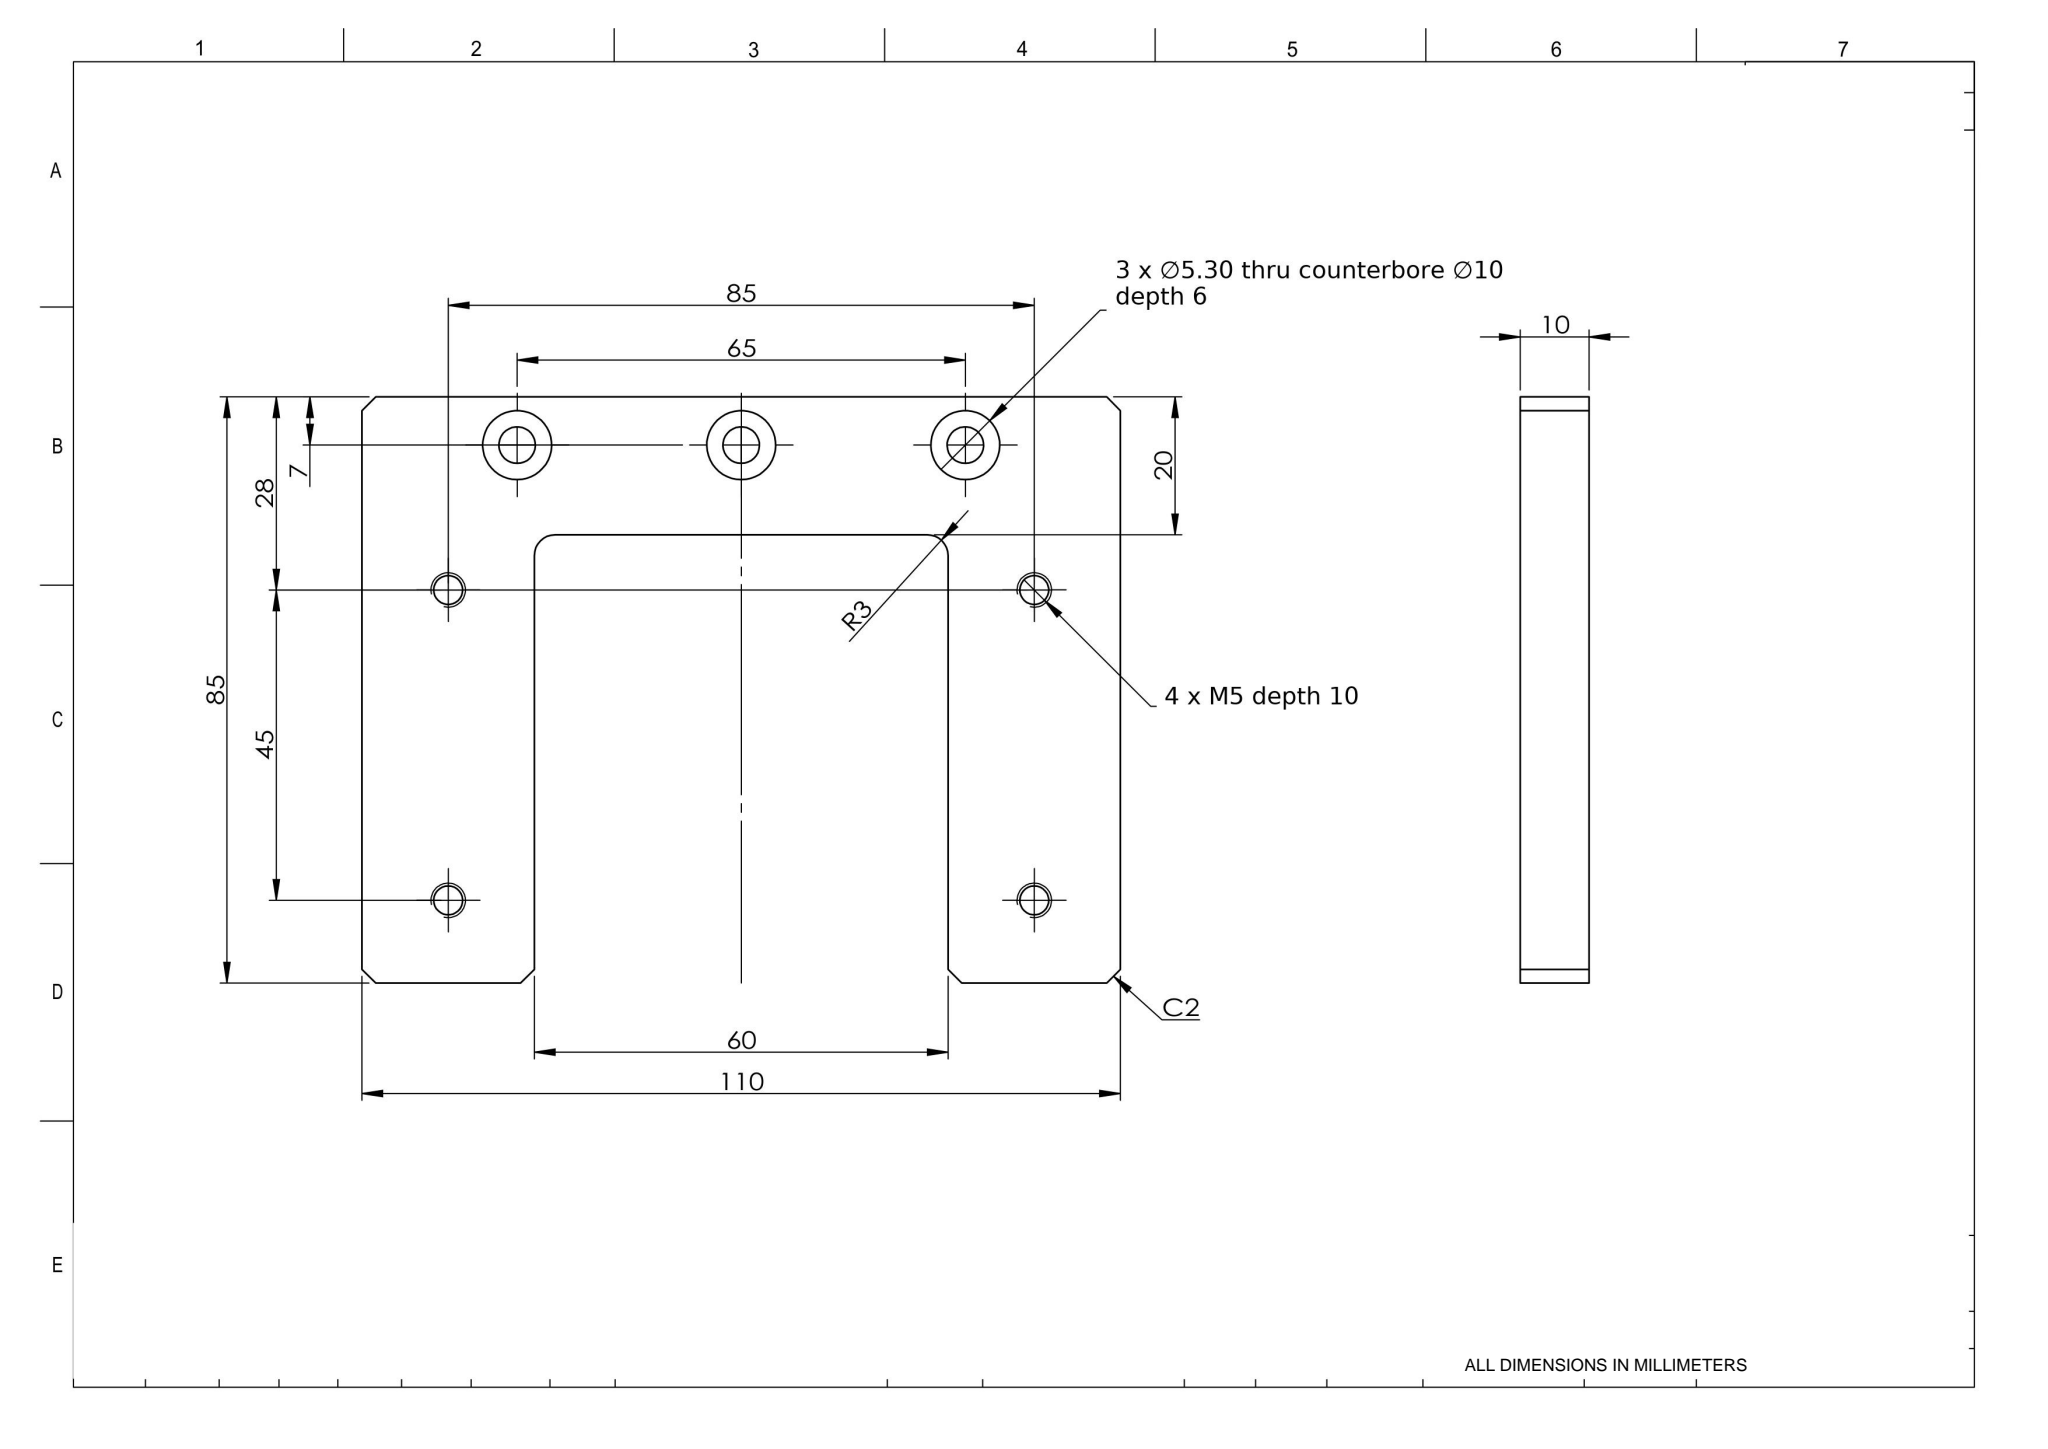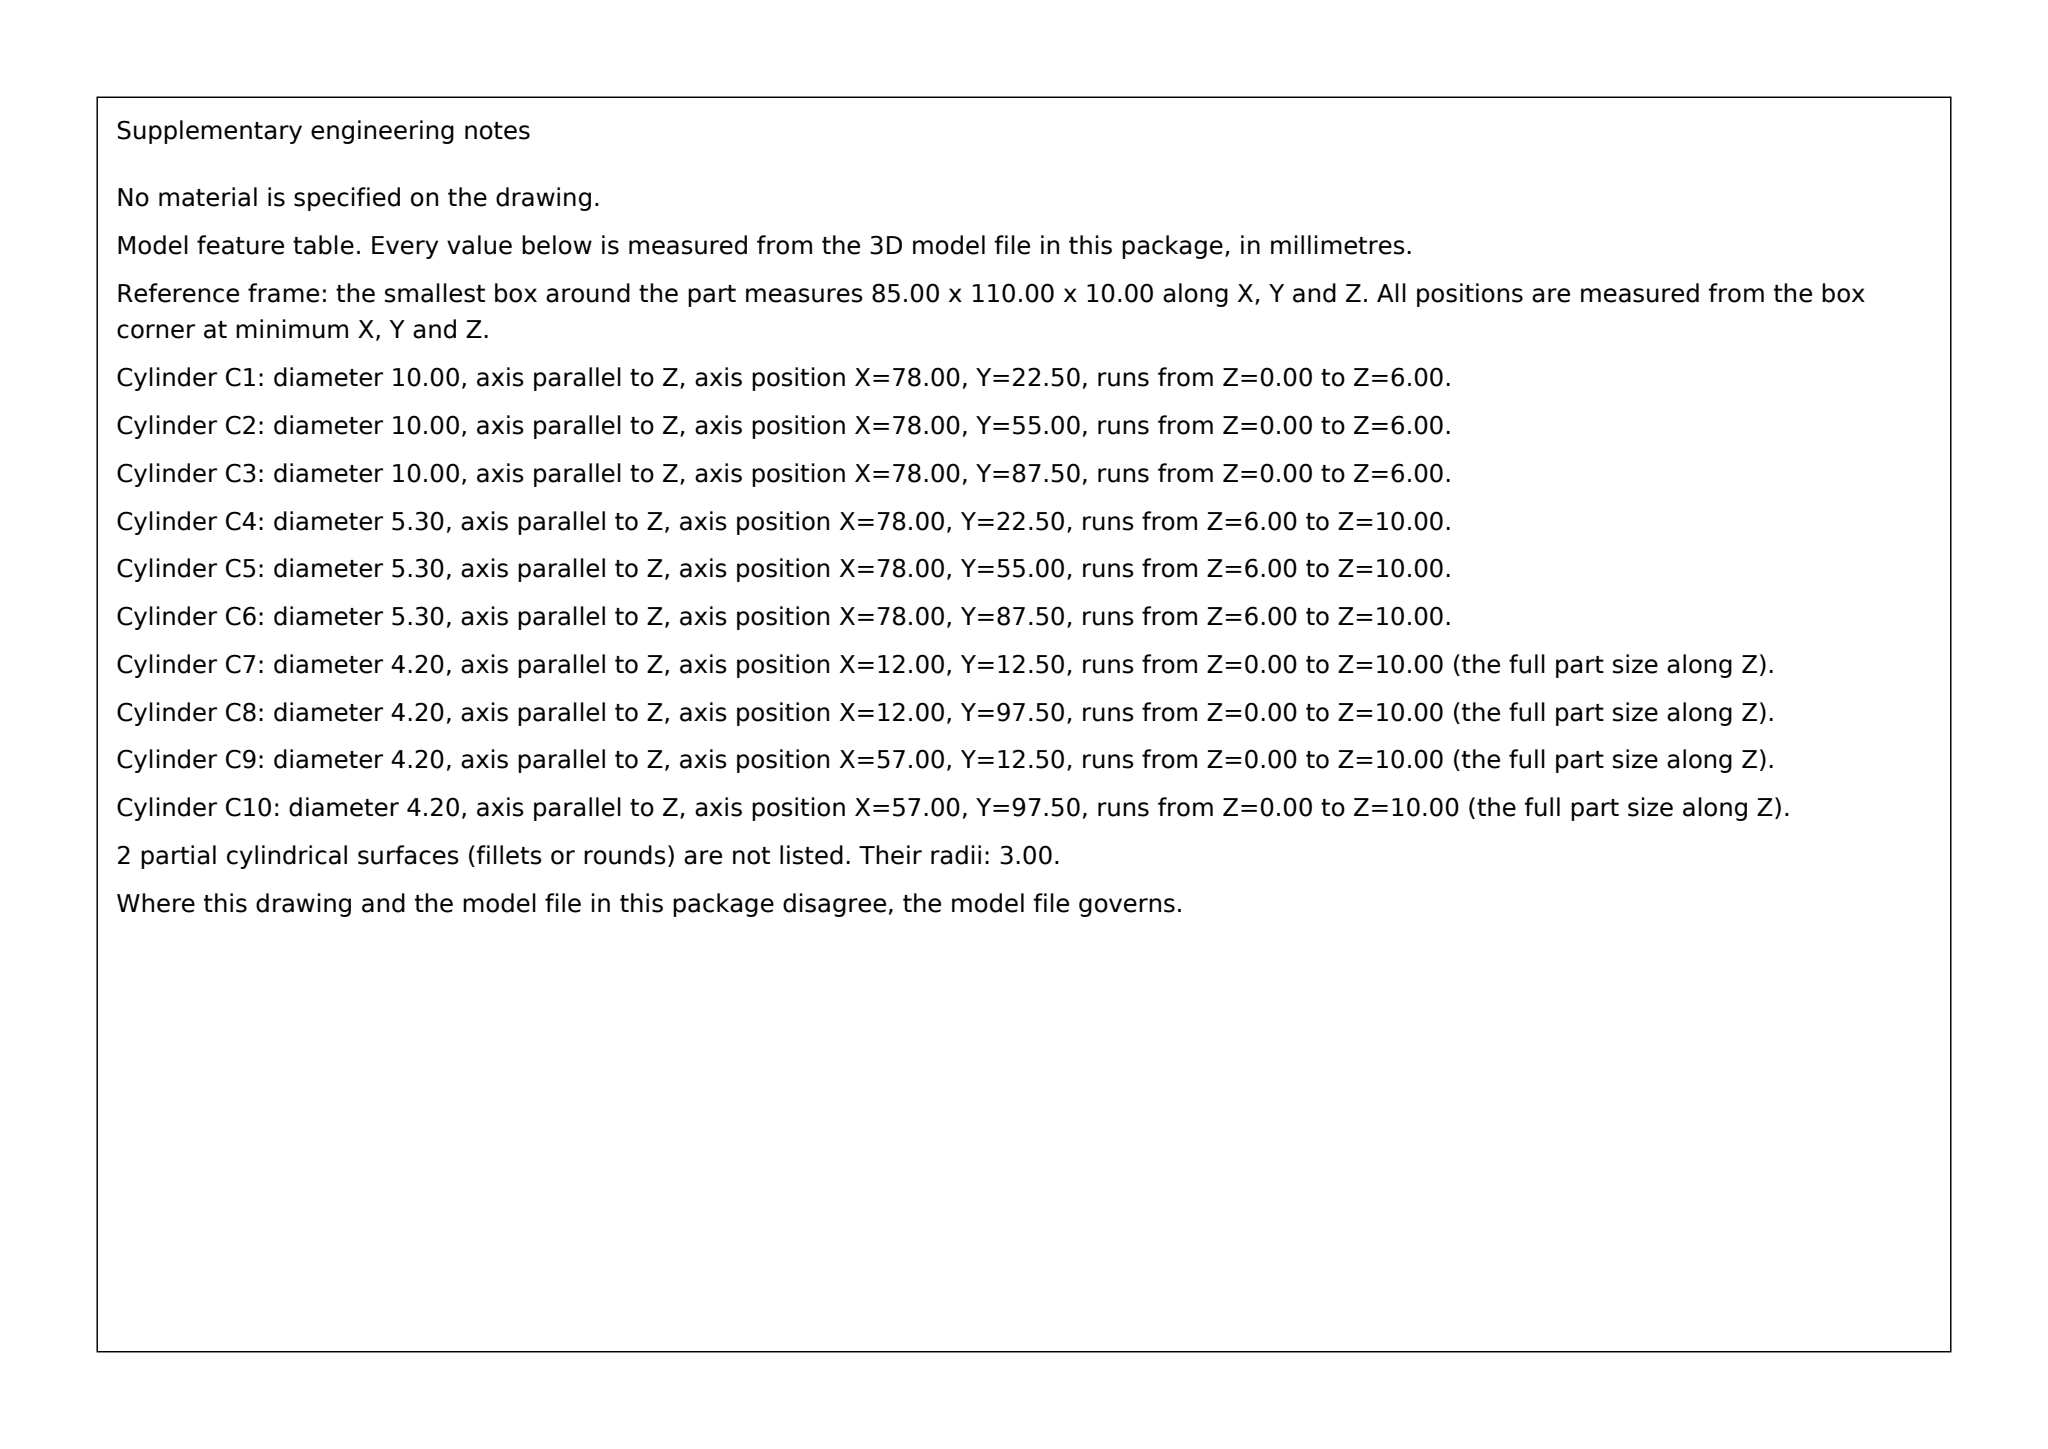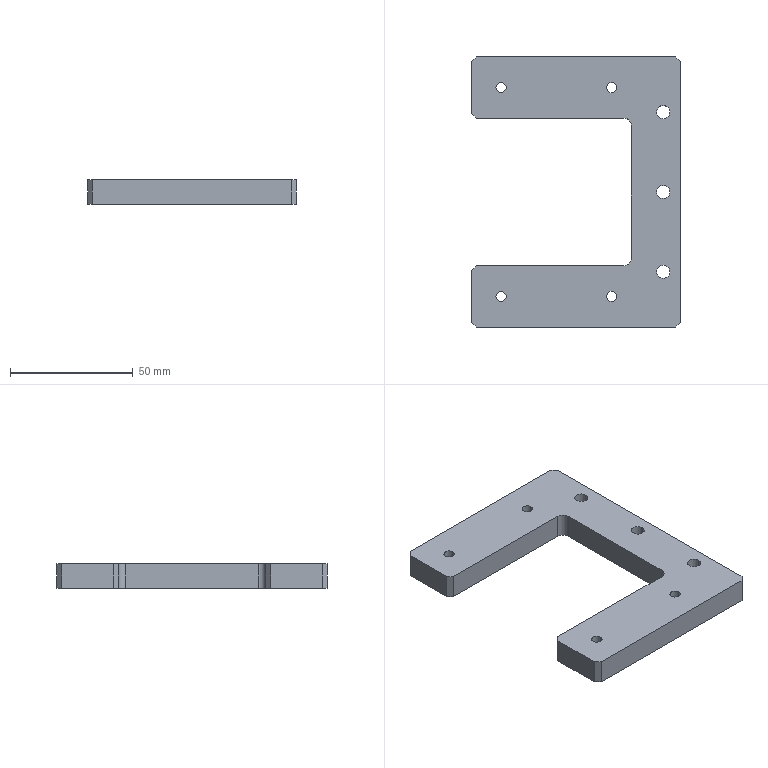Part | SolidWorks | mm | 1 solid | 41 faces | box 85 x 110 x 10 mm | volume 52186 mm3 | cylinder 22 | plane 19 | commonest cylinder face diameters 4.2 x8 10 x6 5.3 x6 6 x2
build123d program:
from build123d import *

# Parameters (mm, degrees)
BOSS_EXTRUDE1_DEPTH                               = 5
FILLET1_R                                         = 3
CHAMFER1_SIZE                                     = 2
M5_TAPPED_HOLE1_D                                 = 4.2
HOLE_SIZE_ACCORDING_TO_HEX_SOCKET_HEA_D           = 5.3
HOLE_SIZE_ACCORDING_TO_HEX_SOCKET_HEA_CBORE_D     = 10
HOLE_SIZE_ACCORDING_TO_HEX_SOCKET_HEA_CBORE_DEPTH = 6


with BuildPart() as part:
    # Sketch1 → Boss-Extrude1 (new, symmetric)
    with BuildSketch(Plane.XY):
        Polygon((0, 55), (0, -55), (-85, -55), (-85, -30), (-20, -30), (-20, 30), (-85, 30), (-85, 55), align=None)
    extrude(amount=BOSS_EXTRUDE1_DEPTH, both=True)

    # Fillet1
    fillet1_edges = [part.edges().sort_by_distance(p)[0] for p in [
        (-20, -30, 0),
        (-20, 30, 0),
    ]]
    fillet(fillet1_edges, radius=FILLET1_R)

    # Chamfer1
    chamfer1_edges = [part.edges().sort_by_distance(p)[0] for p in [
        (0, 55, 0),
        (0, -55, 0),
        (-85, -55, 0),
        (-85, -30, 0),
        (-85, 30, 0),
        (-85, 55, 0),
    ]]
    chamfer(chamfer1_edges, length=CHAMFER1_SIZE)

    # M5 Tapped Hole1 (through all)
    with Locations(Plane.XY.offset(5)):
        with Locations((-28, -42.5), (-73, -42.5), (-73, 42.5), (-28, 42.5)):
            Hole(M5_TAPPED_HOLE1_D / 2)

    # Hole Size _ according to_ Hex Socket Hea (through all)
    with Locations(Plane(origin=(0, 0, -5), x_dir=(-1, 0, 0), z_dir=(0, 0, -1))):
        with Locations((7, -32.5), (7, 0), (7, 32.5)):
            CounterBoreHole(HOLE_SIZE_ACCORDING_TO_HEX_SOCKET_HEA_D / 2, HOLE_SIZE_ACCORDING_TO_HEX_SOCKET_HEA_CBORE_D / 2, HOLE_SIZE_ACCORDING_TO_HEX_SOCKET_HEA_CBORE_DEPTH)


solid = part.part